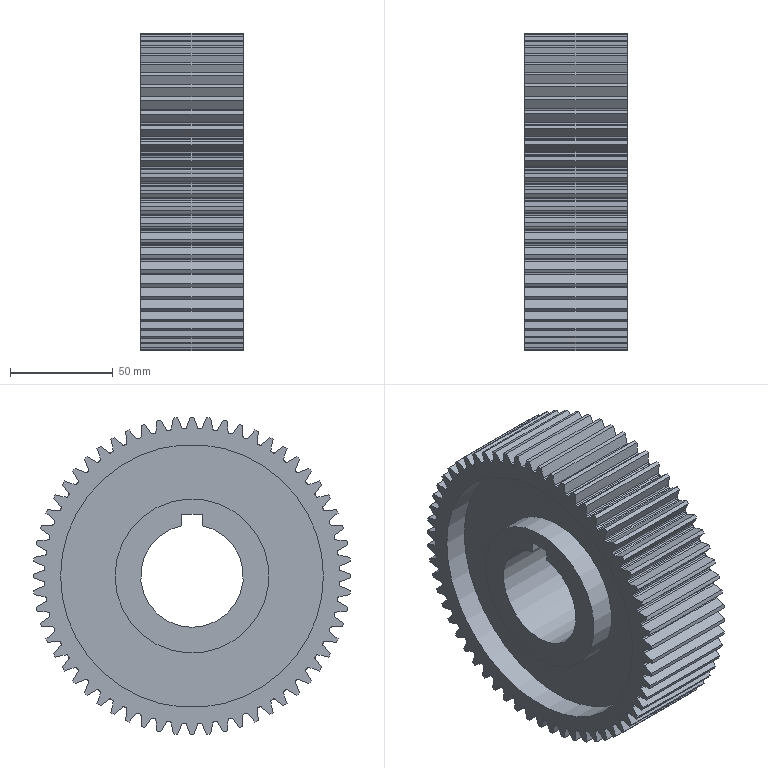Component | NX | SHUCHUZHOUDACHILUN | 1 solid | 374 faces | volume 573199 mm3 | spline 300 | cylinder 65 | plane 9 | commonest cylinder face diameters 143.63 x60 128 x2 75 x2 50 x1